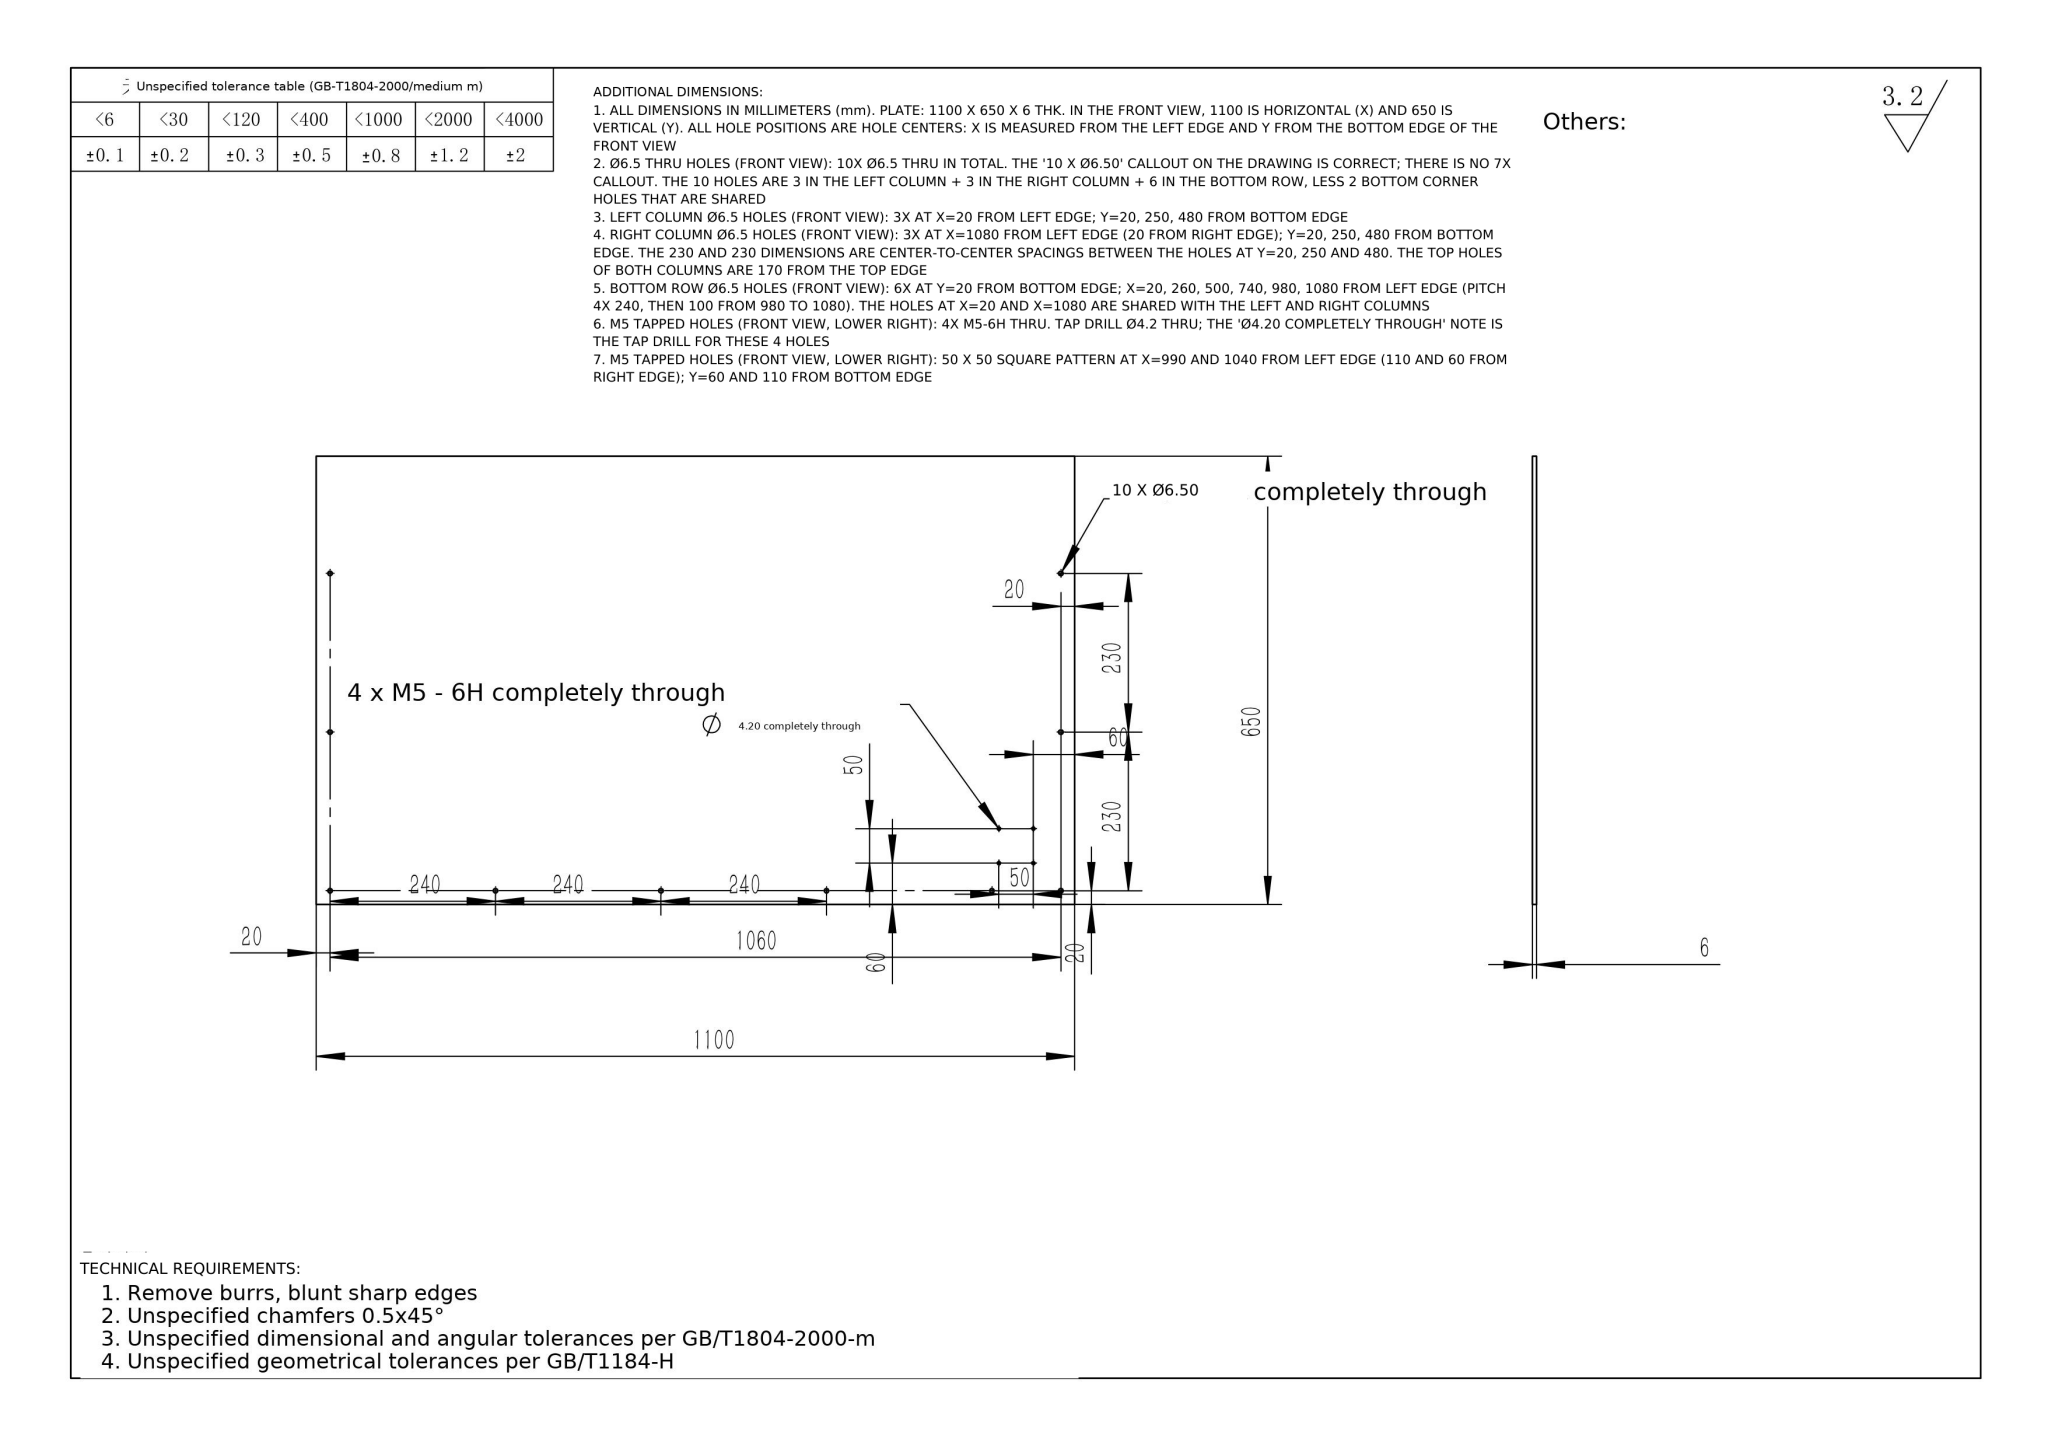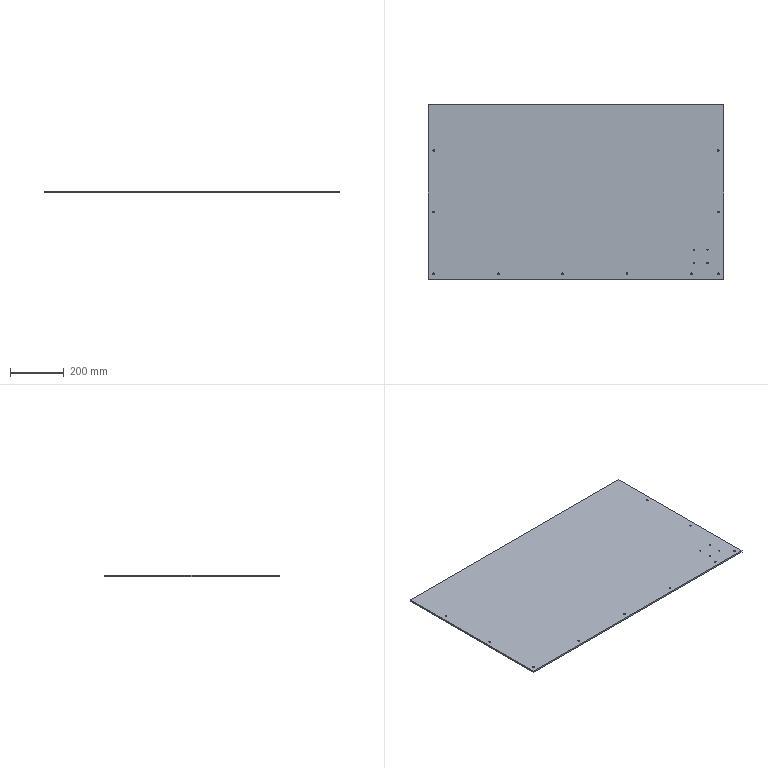Part | NX | mm | 1 solid | 34 faces | box 1100 x 650 x 6 mm | volume 4287677 mm3 | cylinder 28 | plane 6 | commonest cylinder face diameters 6.5 x20 4.2 x8